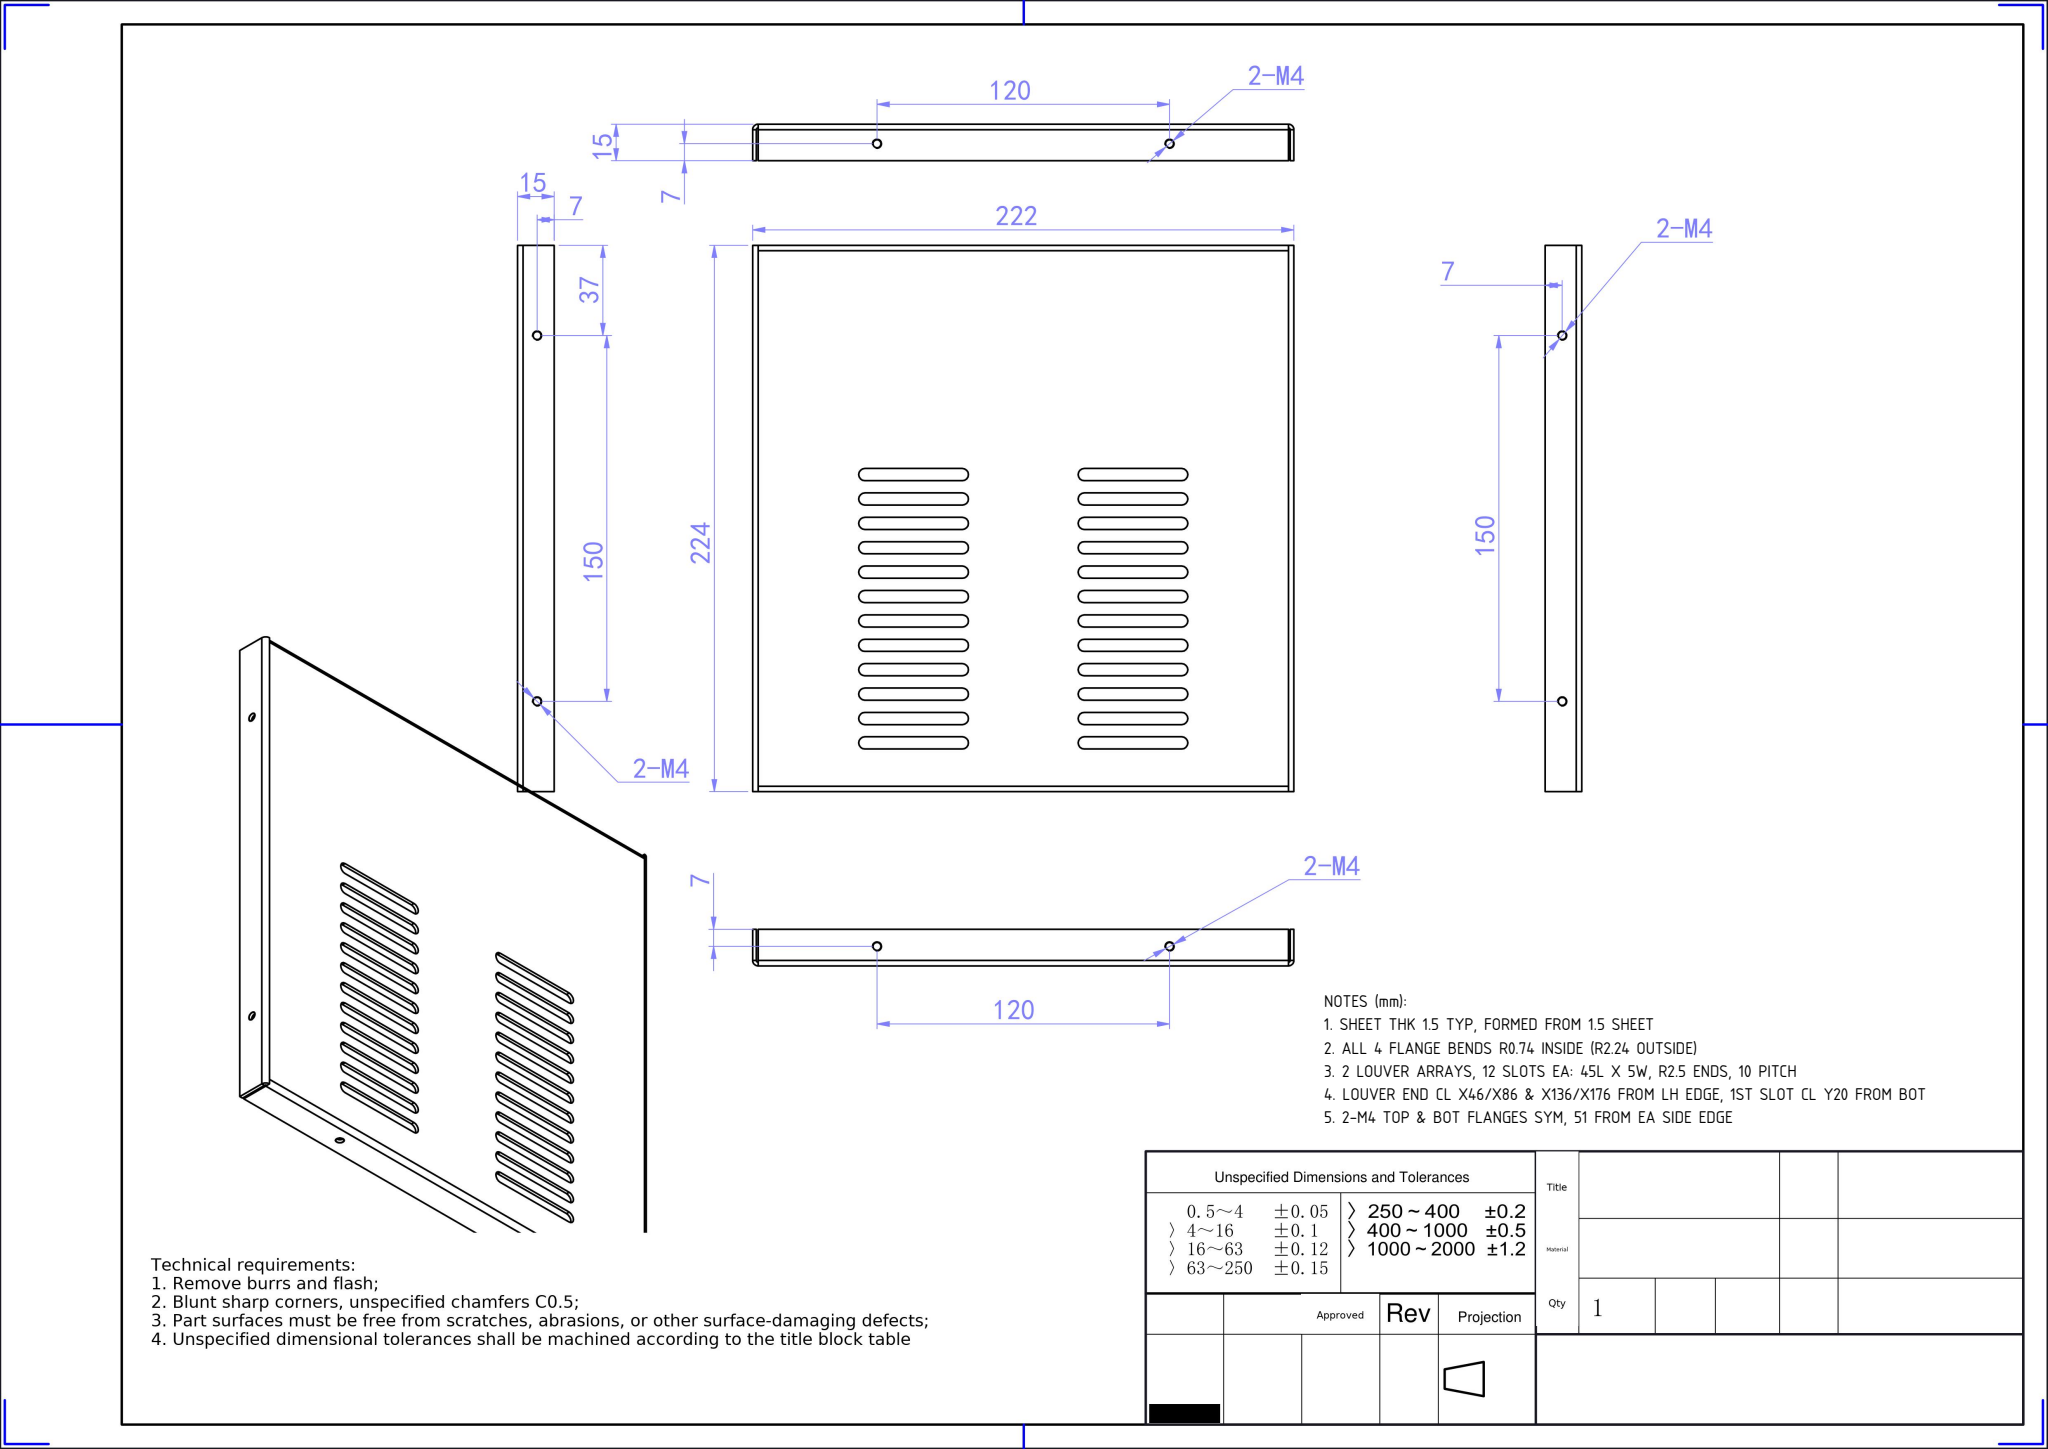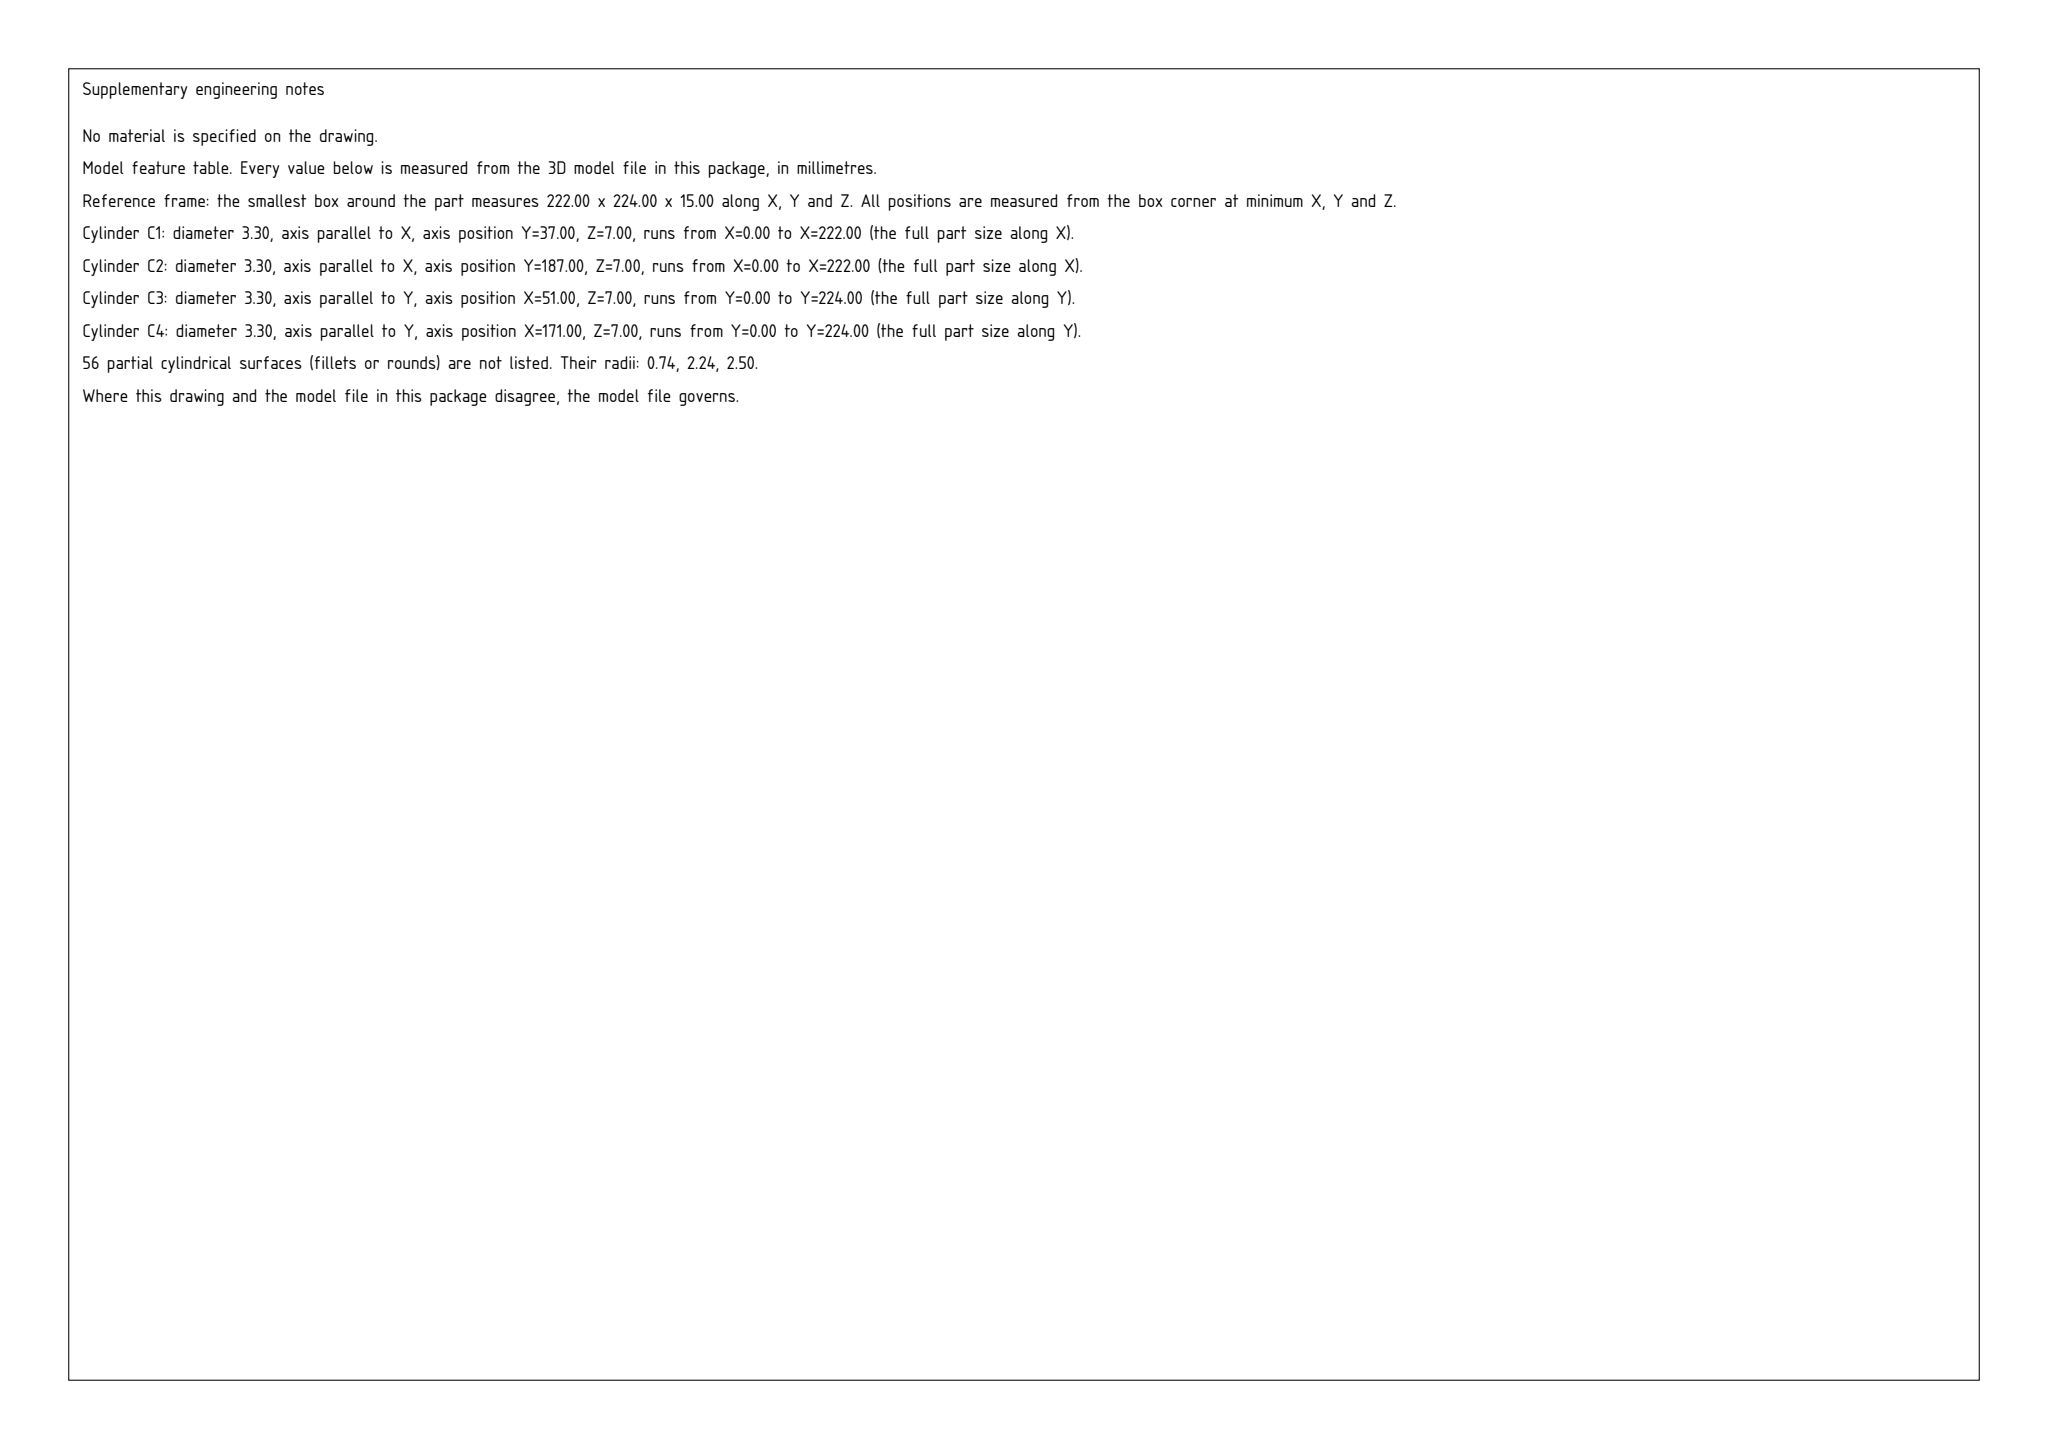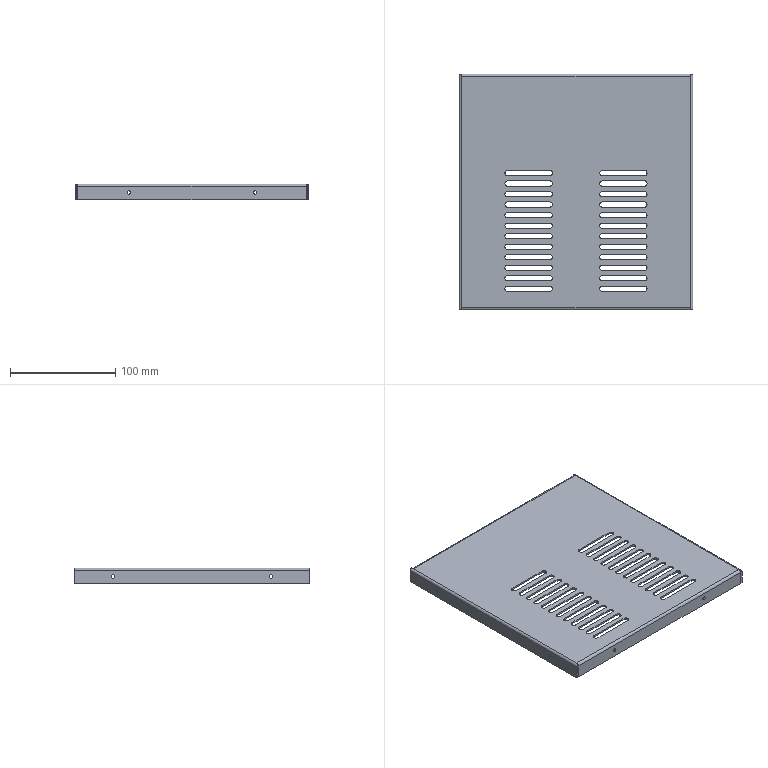Part | SolidWorks | mm | 1 solid | 178 faces | box 222 x 224 x 15 mm | volume 83619 mm3 | cylinder 96 | plane 82 | commonest cylinder face diameters 5 x72 3.3 x16 4.473 x4 1.473 x4
Drawing notes:
SHEET THK 1.5 TYP, FORMED FROM 1.5 SHEET | from the solid: Planes x=0/1.5 & 220.5/222, z=13.5/15 -> wall 1.5
ALL 4 FLANGE BENDS R0.74 INSIDE (R2.24 OUTSIDE) | from the solid: Cyl Ø1.473 (R0.74) & Ø4.473 (R2.24) at x/y=2.24,219.76 & z=12.76, 4 bends
2 LOUVER ARRAYS, 12 SLOTS EA: 45L X 5W, R2.5 ENDS, 10 PITCH | from the solid: Ø5 z-slots, end CL x46-86 & x136-176 (40 apart +5 = 45L); y CL 20..130 step 10
LOUVER END CL X46/X86 & X136/X176 FROM LH EDGE, 1ST SLOT CL Y20 FROM BOT | from the solid: Ø5 cyl pos x=46,86,136,176; y=20 thru 130 from bbox min corner
2-M4 TOP & BOT FLANGES SYM, 51 FROM EA SIDE EDGE | from the solid: Ø3.3 y-axis holes at x=51 and x=171 in 222 wide part, 120 apart